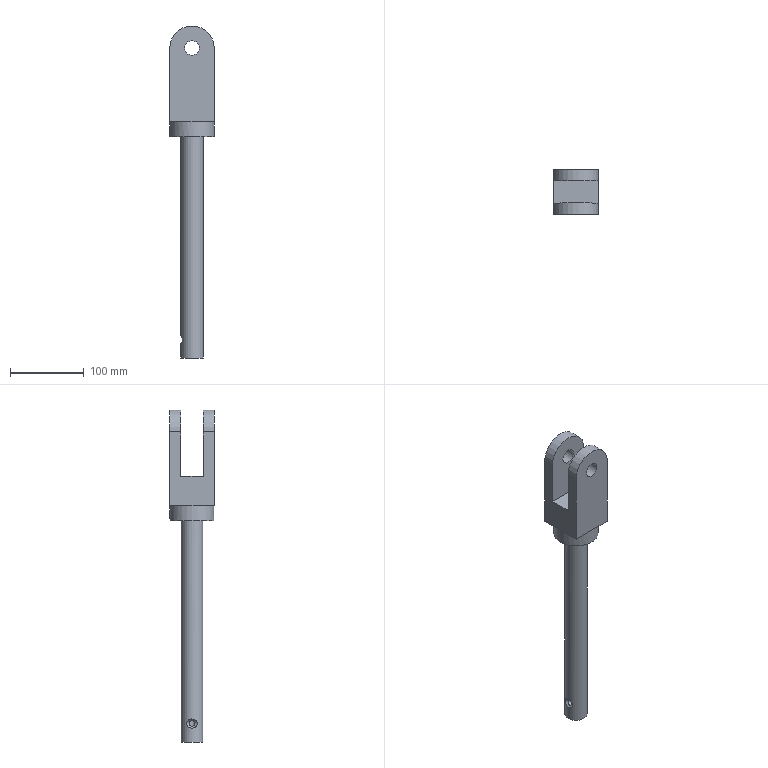Component | NX | PRESSURE_SHAFT | 1 solid | 23 faces | volume 542466 mm3 | plane 14 | cylinder 8 | spline 1 | commonest cylinder face diameters 60 x3 20 x2 30 x1 15 x1 8 x1